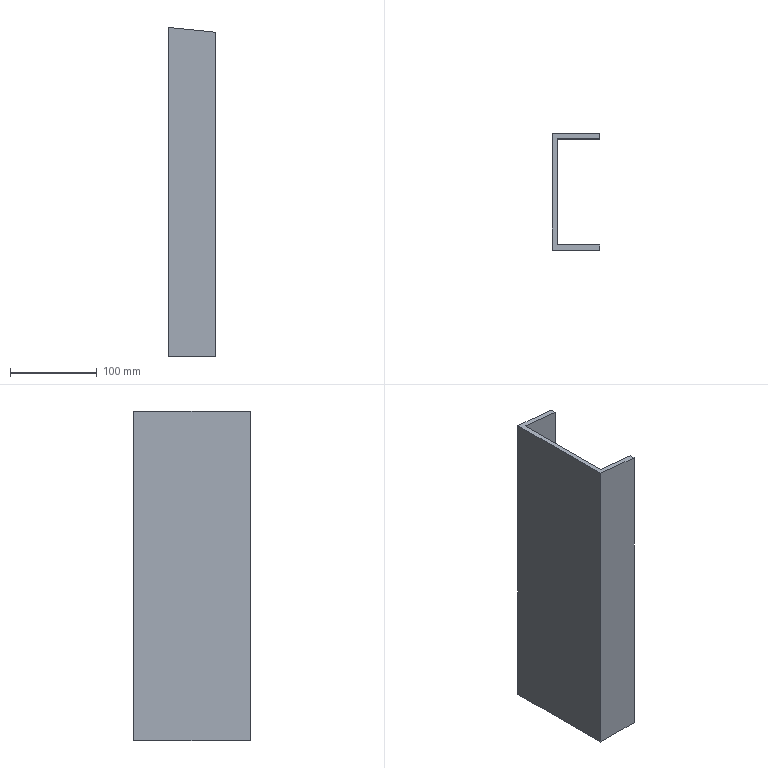Component | NX | RIGHT_FRAME450 | 1 solid | 10 faces | box 55 x 135 x 380.03 mm | volume 529247 mm3 | plane 10
STEP:
#1=CARTESIAN_POINT('',(0.,0.,0.));
#2=DIRECTION('',(0.,0.,1.));
#3=DIRECTION('',(1.,0.,0.));
#4=AXIS2_PLACEMENT_3D('',#1,#2,#3);
#5=CARTESIAN_POINT('',(1375.,1665.,380.029));
#6=VERTEX_POINT('',#5);
#7=CARTESIAN_POINT('',(1375.,1665.,-0.));
#8=VERTEX_POINT('',#7);
#9=CARTESIAN_POINT('',(1375.,1665.,400.));
#10=DIRECTION('',(0.,0.,-1.));
#11=VECTOR('',#10,1.);
#12=LINE('',#9,#11);
#13=CARTESIAN_POINT('',(1375.,1665.,400.));
#14=DIRECTION('',(-1.,0.,0.));
#15=DIRECTION('',(-0.,-1.,0.));
#16=AXIS2_PLACEMENT_3D('',#13,#14,#15);
#17=PLANE('',#16);
#18=CARTESIAN_POINT('',(0.,0.));
#19=DIRECTION('',(0.,-1.));
#20=VECTOR('',#19,1.);
#21=LINE('',#18,#20);
#22=(GEOMETRIC_REPRESENTATION_CONTEXT(2)PARAMETRIC_REPRESENTATION_CONTEXT()REPRESENTATION_CONTEXT('',''));
#23=DEFINITIONAL_REPRESENTATION('',(#21),#22);
#24=PCURVE('',#17,#23);
#25=CARTESIAN_POINT('',(1430.,1665.,400.));
#26=DIRECTION('',(0.,-1.,0.));
#27=DIRECTION('',(0.,0.,-1.));
#28=AXIS2_PLACEMENT_3D('',#25,#26,#27);
#29=PLANE('',#28);
#30=CARTESIAN_POINT('',(0.,-55.));
#31=DIRECTION('',(1.,0.));
#32=VECTOR('',#31,1.);
#33=LINE('',#30,#32);
#34=(GEOMETRIC_REPRESENTATION_CONTEXT(2)PARAMETRIC_REPRESENTATION_CONTEXT()REPRESENTATION_CONTEXT('',''));
#35=DEFINITIONAL_REPRESENTATION('',(#33),#34);
#36=PCURVE('',#29,#35);
#37=SURFACE_CURVE('',#12,(#24,#36),.PCURVE_S1.);
#38=EDGE_CURVE('',#6,#8,#37,.T.);
#39=ORIENTED_EDGE('',*,*,#38,.F.);
#40=CARTESIAN_POINT('',(1375.,1800.,380.029));
#41=VERTEX_POINT('',#40);
#42=CARTESIAN_POINT('',(1375.,1665.,380.029));
#43=DIRECTION('',(0.,1.,-0.));
#44=VECTOR('',#43,1.);
#45=LINE('',#42,#44);
#46=CARTESIAN_POINT('',(0.,-19.971));
#47=DIRECTION('',(-1.,-0.));
#48=VECTOR('',#47,1.);
#49=LINE('',#46,#48);
#50=(GEOMETRIC_REPRESENTATION_CONTEXT(2)PARAMETRIC_REPRESENTATION_CONTEXT()REPRESENTATION_CONTEXT('',''));
#51=DEFINITIONAL_REPRESENTATION('',(#49),#50);
#52=PCURVE('',#17,#51);
#53=CARTESIAN_POINT('',(1470.271,2035.,370.519));
#54=DIRECTION('',(0.09932,0.,0.9951));
#55=DIRECTION('',(0.9951,0.,-0.09932));
#56=AXIS2_PLACEMENT_3D('',#53,#54,#55);
#57=PLANE('',#56);
#58=CARTESIAN_POINT('',(-95.744,-370.));
#59=DIRECTION('',(0.,1.));
#60=VECTOR('',#59,1.);
#61=LINE('',#58,#60);
#62=(GEOMETRIC_REPRESENTATION_CONTEXT(2)PARAMETRIC_REPRESENTATION_CONTEXT()REPRESENTATION_CONTEXT('',''));
#63=DEFINITIONAL_REPRESENTATION('',(#61),#62);
#64=PCURVE('',#57,#63);
#65=SURFACE_CURVE('',#45,(#52,#64),.PCURVE_S1.);
#66=EDGE_CURVE('',#6,#41,#65,.T.);
#67=ORIENTED_EDGE('',*,*,#66,.T.);
#68=CARTESIAN_POINT('',(1375.,1800.,-0.));
#69=VERTEX_POINT('',#68);
#70=CARTESIAN_POINT('',(1375.,1800.,400.));
#71=DIRECTION('',(0.,0.,-1.));
#72=VECTOR('',#71,1.);
#73=LINE('',#70,#72);
#74=CARTESIAN_POINT('',(-135.,0.));
#75=DIRECTION('',(0.,-1.));
#76=VECTOR('',#75,1.);
#77=LINE('',#74,#76);
#78=(GEOMETRIC_REPRESENTATION_CONTEXT(2)PARAMETRIC_REPRESENTATION_CONTEXT()REPRESENTATION_CONTEXT('',''));
#79=DEFINITIONAL_REPRESENTATION('',(#77),#78);
#80=PCURVE('',#17,#79);
#81=CARTESIAN_POINT('',(1375.,1800.,400.));
#82=DIRECTION('',(0.,1.,0.));
#83=DIRECTION('',(0.,0.,1.));
#84=AXIS2_PLACEMENT_3D('',#81,#82,#83);
#85=PLANE('',#84);
#86=CARTESIAN_POINT('',(0.,0.));
#87=DIRECTION('',(-1.,0.));
#88=VECTOR('',#87,1.);
#89=LINE('',#86,#88);
#90=(GEOMETRIC_REPRESENTATION_CONTEXT(2)PARAMETRIC_REPRESENTATION_CONTEXT()REPRESENTATION_CONTEXT('',''));
#91=DEFINITIONAL_REPRESENTATION('',(#89),#90);
#92=PCURVE('',#85,#91);
#93=SURFACE_CURVE('',#73,(#80,#92),.PCURVE_S1.);
#94=EDGE_CURVE('',#41,#69,#93,.T.);
#95=ORIENTED_EDGE('',*,*,#94,.T.);
#96=CARTESIAN_POINT('',(1375.,1665.,-0.));
#97=DIRECTION('',(0.,1.,0.));
#98=VECTOR('',#97,1.);
#99=LINE('',#96,#98);
#100=CARTESIAN_POINT('',(0.,-400.));
#101=DIRECTION('',(-1.,0.));
#102=VECTOR('',#101,1.);
#103=LINE('',#100,#102);
#104=(GEOMETRIC_REPRESENTATION_CONTEXT(2)PARAMETRIC_REPRESENTATION_CONTEXT()REPRESENTATION_CONTEXT('',''));
#105=DEFINITIONAL_REPRESENTATION('',(#103),#104);
#106=PCURVE('',#17,#105);
#107=CARTESIAN_POINT('',(1375.,1800.,-0.));
#108=DIRECTION('',(0.,0.,-1.));
#109=DIRECTION('',(-1.,0.,0.));
#110=AXIS2_PLACEMENT_3D('',#107,#108,#109);
#111=PLANE('',#110);
#112=CARTESIAN_POINT('',(0.,-135.));
#113=DIRECTION('',(-0.,1.));
#114=VECTOR('',#113,1.);
#115=LINE('',#112,#114);
#116=(GEOMETRIC_REPRESENTATION_CONTEXT(2)PARAMETRIC_REPRESENTATION_CONTEXT()REPRESENTATION_CONTEXT('',''));
#117=DEFINITIONAL_REPRESENTATION('',(#115),#116);
#118=PCURVE('',#111,#117);
#119=SURFACE_CURVE('',#99,(#106,#118),.PCURVE_S1.);
#120=EDGE_CURVE('',#8,#69,#119,.T.);
#121=ORIENTED_EDGE('',*,*,#120,.F.);
#122=EDGE_LOOP('',(#39,#67,#95,#121));
#123=FACE_BOUND('',#122,.T.);
#124=ADVANCED_FACE('',(#123),#17,.T.);
#125=ORIENTED_EDGE('',*,*,#94,.F.);
#126=CARTESIAN_POINT('',(1430.,1800.,374.539));
#127=VERTEX_POINT('',#126);
#128=CARTESIAN_POINT('',(1373.026,1800.,380.226));
#129=DIRECTION('',(0.9951,0.,-0.09932));
#130=VECTOR('',#129,1.);
#131=LINE('',#128,#130);
#132=CARTESIAN_POINT('',(-19.774,-1.974));
#133=DIRECTION('',(-0.09932,0.9951));
#134=VECTOR('',#133,1.);
#135=LINE('',#132,#134);
#136=(GEOMETRIC_REPRESENTATION_CONTEXT(2)PARAMETRIC_REPRESENTATION_CONTEXT()REPRESENTATION_CONTEXT('',''));
#137=DEFINITIONAL_REPRESENTATION('',(#135),#136);
#138=PCURVE('',#85,#137);
#139=CARTESIAN_POINT('',(-97.728,-235.));
#140=DIRECTION('',(1.,0.));
#141=VECTOR('',#140,1.);
#142=LINE('',#139,#141);
#143=(GEOMETRIC_REPRESENTATION_CONTEXT(2)PARAMETRIC_REPRESENTATION_CONTEXT()REPRESENTATION_CONTEXT('',''));
#144=DEFINITIONAL_REPRESENTATION('',(#142),#143);
#145=PCURVE('',#57,#144);
#146=SURFACE_CURVE('',#131,(#138,#145),.PCURVE_S1.);
#147=EDGE_CURVE('',#41,#127,#146,.T.);
#148=ORIENTED_EDGE('',*,*,#147,.T.);
#149=CARTESIAN_POINT('',(1430.,1800.,-0.));
#150=VERTEX_POINT('',#149);
#151=CARTESIAN_POINT('',(1430.,1800.,400.));
#152=DIRECTION('',(0.,0.,-1.));
#153=VECTOR('',#152,1.);
#154=LINE('',#151,#153);
#155=CARTESIAN_POINT('',(0.,55.));
#156=DIRECTION('',(-1.,0.));
#157=VECTOR('',#156,1.);
#158=LINE('',#155,#157);
#159=(GEOMETRIC_REPRESENTATION_CONTEXT(2)PARAMETRIC_REPRESENTATION_CONTEXT()REPRESENTATION_CONTEXT('',''));
#160=DEFINITIONAL_REPRESENTATION('',(#158),#159);
#161=PCURVE('',#85,#160);
#162=CARTESIAN_POINT('',(1430.,1800.,400.));
#163=DIRECTION('',(1.,-0.,0.));
#164=DIRECTION('',(0.,1.,0.));
#165=AXIS2_PLACEMENT_3D('',#162,#163,#164);
#166=PLANE('',#165);
#167=CARTESIAN_POINT('',(0.,0.));
#168=DIRECTION('',(0.,-1.));
#169=VECTOR('',#168,1.);
#170=LINE('',#167,#169);
#171=(GEOMETRIC_REPRESENTATION_CONTEXT(2)PARAMETRIC_REPRESENTATION_CONTEXT()REPRESENTATION_CONTEXT('',''));
#172=DEFINITIONAL_REPRESENTATION('',(#170),#171);
#173=PCURVE('',#166,#172);
#174=SURFACE_CURVE('',#154,(#161,#173),.PCURVE_S1.);
#175=EDGE_CURVE('',#127,#150,#174,.T.);
#176=ORIENTED_EDGE('',*,*,#175,.T.);
#177=CARTESIAN_POINT('',(1375.,1800.,-0.));
#178=DIRECTION('',(1.,0.,0.));
#179=VECTOR('',#178,1.);
#180=LINE('',#177,#179);
#181=CARTESIAN_POINT('',(-400.,0.));
#182=DIRECTION('',(0.,1.));
#183=VECTOR('',#182,1.);
#184=LINE('',#181,#183);
#185=(GEOMETRIC_REPRESENTATION_CONTEXT(2)PARAMETRIC_REPRESENTATION_CONTEXT()REPRESENTATION_CONTEXT('',''));
#186=DEFINITIONAL_REPRESENTATION('',(#184),#185);
#187=PCURVE('',#85,#186);
#188=CARTESIAN_POINT('',(0.,0.));
#189=DIRECTION('',(-1.,0.));
#190=VECTOR('',#189,1.);
#191=LINE('',#188,#190);
#192=(GEOMETRIC_REPRESENTATION_CONTEXT(2)PARAMETRIC_REPRESENTATION_CONTEXT()REPRESENTATION_CONTEXT('',''));
#193=DEFINITIONAL_REPRESENTATION('',(#191),#192);
#194=PCURVE('',#111,#193);
#195=SURFACE_CURVE('',#180,(#187,#194),.PCURVE_S1.);
#196=EDGE_CURVE('',#69,#150,#195,.T.);
#197=ORIENTED_EDGE('',*,*,#196,.F.);
#198=EDGE_LOOP('',(#125,#148,#176,#197));
#199=FACE_BOUND('',#198,.T.);
#200=ADVANCED_FACE('',(#199),#85,.T.);
#201=ORIENTED_EDGE('',*,*,#175,.F.);
#202=CARTESIAN_POINT('',(1430.,1794.,374.539));
#203=VERTEX_POINT('',#202);
#204=CARTESIAN_POINT('',(1430.,1800.,374.539));
#205=DIRECTION('',(-0.,-1.,0.));
#206=VECTOR('',#205,1.);
#207=LINE('',#204,#206);
#208=CARTESIAN_POINT('',(0.,-25.461));
#209=DIRECTION('',(-1.,0.));
#210=VECTOR('',#209,1.);
#211=LINE('',#208,#210);
#212=(GEOMETRIC_REPRESENTATION_CONTEXT(2)PARAMETRIC_REPRESENTATION_CONTEXT()REPRESENTATION_CONTEXT('',''));
#213=DEFINITIONAL_REPRESENTATION('',(#211),#212);
#214=PCURVE('',#166,#213);
#215=CARTESIAN_POINT('',(-40.471,-235.));
#216=DIRECTION('',(-0.,-1.));
#217=VECTOR('',#216,1.);
#218=LINE('',#215,#217);
#219=(GEOMETRIC_REPRESENTATION_CONTEXT(2)PARAMETRIC_REPRESENTATION_CONTEXT()REPRESENTATION_CONTEXT('',''));
#220=DEFINITIONAL_REPRESENTATION('',(#218),#219);
#221=PCURVE('',#57,#220);
#222=SURFACE_CURVE('',#207,(#214,#221),.PCURVE_S1.);
#223=EDGE_CURVE('',#127,#203,#222,.T.);
#224=ORIENTED_EDGE('',*,*,#223,.T.);
#225=CARTESIAN_POINT('',(1430.,1794.,-0.));
#226=VERTEX_POINT('',#225);
#227=CARTESIAN_POINT('',(1430.,1794.,400.));
#228=DIRECTION('',(0.,0.,-1.));
#229=VECTOR('',#228,1.);
#230=LINE('',#227,#229);
#231=CARTESIAN_POINT('',(-6.,0.));
#232=DIRECTION('',(0.,-1.));
#233=VECTOR('',#232,1.);
#234=LINE('',#231,#233);
#235=(GEOMETRIC_REPRESENTATION_CONTEXT(2)PARAMETRIC_REPRESENTATION_CONTEXT()REPRESENTATION_CONTEXT('',''));
#236=DEFINITIONAL_REPRESENTATION('',(#234),#235);
#237=PCURVE('',#166,#236);
#238=CARTESIAN_POINT('',(1430.,1794.,400.));
#239=DIRECTION('',(-0.,-1.,0.));
#240=DIRECTION('',(1.,-0.,0.));
#241=AXIS2_PLACEMENT_3D('',#238,#239,#240);
#242=PLANE('',#241);
#243=CARTESIAN_POINT('',(0.,0.));
#244=DIRECTION('',(0.,-1.));
#245=VECTOR('',#244,1.);
#246=LINE('',#243,#245);
#247=(GEOMETRIC_REPRESENTATION_CONTEXT(2)PARAMETRIC_REPRESENTATION_CONTEXT()REPRESENTATION_CONTEXT('',''));
#248=DEFINITIONAL_REPRESENTATION('',(#246),#247);
#249=PCURVE('',#242,#248);
#250=SURFACE_CURVE('',#230,(#237,#249),.PCURVE_S1.);
#251=EDGE_CURVE('',#203,#226,#250,.T.);
#252=ORIENTED_EDGE('',*,*,#251,.T.);
#253=CARTESIAN_POINT('',(1430.,1800.,-0.));
#254=DIRECTION('',(-0.,-1.,0.));
#255=VECTOR('',#254,1.);
#256=LINE('',#253,#255);
#257=CARTESIAN_POINT('',(0.,-400.));
#258=DIRECTION('',(-1.,0.));
#259=VECTOR('',#258,1.);
#260=LINE('',#257,#259);
#261=(GEOMETRIC_REPRESENTATION_CONTEXT(2)PARAMETRIC_REPRESENTATION_CONTEXT()REPRESENTATION_CONTEXT('',''));
#262=DEFINITIONAL_REPRESENTATION('',(#260),#261);
#263=PCURVE('',#166,#262);
#264=CARTESIAN_POINT('',(-55.,0.));
#265=DIRECTION('',(0.,-1.));
#266=VECTOR('',#265,1.);
#267=LINE('',#264,#266);
#268=(GEOMETRIC_REPRESENTATION_CONTEXT(2)PARAMETRIC_REPRESENTATION_CONTEXT()REPRESENTATION_CONTEXT('',''));
#269=DEFINITIONAL_REPRESENTATION('',(#267),#268);
#270=PCURVE('',#111,#269);
#271=SURFACE_CURVE('',#256,(#263,#270),.PCURVE_S1.);
#272=EDGE_CURVE('',#150,#226,#271,.T.);
#273=ORIENTED_EDGE('',*,*,#272,.F.);
#274=EDGE_LOOP('',(#201,#224,#252,#273));
#275=FACE_BOUND('',#274,.T.);
#276=ADVANCED_FACE('',(#275),#166,.T.);
#277=ORIENTED_EDGE('',*,*,#251,.F.);
#278=CARTESIAN_POINT('',(1381.,1794.,379.43));
#279=VERTEX_POINT('',#278);
#280=CARTESIAN_POINT('',(1427.484,1794.,374.79));
#281=DIRECTION('',(-0.9951,0.,0.09932));
#282=VECTOR('',#281,1.);
#283=LINE('',#280,#282);
#284=CARTESIAN_POINT('',(-2.516,-25.21));
#285=DIRECTION('',(-0.9951,0.09932));
#286=VECTOR('',#285,1.);
#287=LINE('',#284,#286);
#288=(GEOMETRIC_REPRESENTATION_CONTEXT(2)PARAMETRIC_REPRESENTATION_CONTEXT()REPRESENTATION_CONTEXT('',''));
#289=DEFINITIONAL_REPRESENTATION('',(#287),#288);
#290=PCURVE('',#242,#289);
#291=CARTESIAN_POINT('',(-43.,-241.));
#292=DIRECTION('',(-1.,0.));
#293=VECTOR('',#292,1.);
#294=LINE('',#291,#293);
#295=(GEOMETRIC_REPRESENTATION_CONTEXT(2)PARAMETRIC_REPRESENTATION_CONTEXT()REPRESENTATION_CONTEXT('',''));
#296=DEFINITIONAL_REPRESENTATION('',(#294),#295);
#297=PCURVE('',#57,#296);
#298=SURFACE_CURVE('',#283,(#290,#297),.PCURVE_S1.);
#299=EDGE_CURVE('',#203,#279,#298,.T.);
#300=ORIENTED_EDGE('',*,*,#299,.T.);
#301=CARTESIAN_POINT('',(1381.,1794.,-0.));
#302=VERTEX_POINT('',#301);
#303=CARTESIAN_POINT('',(1381.,1794.,400.));
#304=DIRECTION('',(0.,0.,-1.));
#305=VECTOR('',#304,1.);
#306=LINE('',#303,#305);
#307=CARTESIAN_POINT('',(-49.,0.));
#308=DIRECTION('',(0.,-1.));
#309=VECTOR('',#308,1.);
#310=LINE('',#307,#309);
#311=(GEOMETRIC_REPRESENTATION_CONTEXT(2)PARAMETRIC_REPRESENTATION_CONTEXT()REPRESENTATION_CONTEXT('',''));
#312=DEFINITIONAL_REPRESENTATION('',(#310),#311);
#313=PCURVE('',#242,#312);
#314=CARTESIAN_POINT('',(1381.,1794.,400.));
#315=DIRECTION('',(1.,-0.,0.));
#316=DIRECTION('',(0.,1.,0.));
#317=AXIS2_PLACEMENT_3D('',#314,#315,#316);
#318=PLANE('',#317);
#319=CARTESIAN_POINT('',(0.,0.));
#320=DIRECTION('',(0.,-1.));
#321=VECTOR('',#320,1.);
#322=LINE('',#319,#321);
#323=(GEOMETRIC_REPRESENTATION_CONTEXT(2)PARAMETRIC_REPRESENTATION_CONTEXT()REPRESENTATION_CONTEXT('',''));
#324=DEFINITIONAL_REPRESENTATION('',(#322),#323);
#325=PCURVE('',#318,#324);
#326=SURFACE_CURVE('',#306,(#313,#325),.PCURVE_S1.);
#327=EDGE_CURVE('',#279,#302,#326,.T.);
#328=ORIENTED_EDGE('',*,*,#327,.T.);
#329=CARTESIAN_POINT('',(1430.,1794.,-0.));
#330=DIRECTION('',(-1.,0.,0.));
#331=VECTOR('',#330,1.);
#332=LINE('',#329,#331);
#333=CARTESIAN_POINT('',(0.,-400.));
#334=DIRECTION('',(-1.,0.));
#335=VECTOR('',#334,1.);
#336=LINE('',#333,#335);
#337=(GEOMETRIC_REPRESENTATION_CONTEXT(2)PARAMETRIC_REPRESENTATION_CONTEXT()REPRESENTATION_CONTEXT('',''));
#338=DEFINITIONAL_REPRESENTATION('',(#336),#337);
#339=PCURVE('',#242,#338);
#340=CARTESIAN_POINT('',(-55.,-6.));
#341=DIRECTION('',(1.,0.));
#342=VECTOR('',#341,1.);
#343=LINE('',#340,#342);
#344=(GEOMETRIC_REPRESENTATION_CONTEXT(2)PARAMETRIC_REPRESENTATION_CONTEXT()REPRESENTATION_CONTEXT('',''));
#345=DEFINITIONAL_REPRESENTATION('',(#343),#344);
#346=PCURVE('',#111,#345);
#347=SURFACE_CURVE('',#332,(#339,#346),.PCURVE_S1.);
#348=EDGE_CURVE('',#226,#302,#347,.T.);
#349=ORIENTED_EDGE('',*,*,#348,.F.);
#350=EDGE_LOOP('',(#277,#300,#328,#349));
#351=FACE_BOUND('',#350,.T.);
#352=ADVANCED_FACE('',(#351),#242,.T.);
#353=ORIENTED_EDGE('',*,*,#327,.F.);
#354=CARTESIAN_POINT('',(1381.,1671.,379.43));
#355=VERTEX_POINT('',#354);
#356=CARTESIAN_POINT('',(1381.,1794.,379.43));
#357=DIRECTION('',(-0.,-1.,0.));
#358=VECTOR('',#357,1.);
#359=LINE('',#356,#358);
#360=CARTESIAN_POINT('',(0.,-20.57));
#361=DIRECTION('',(-1.,0.));
#362=VECTOR('',#361,1.);
#363=LINE('',#360,#362);
#364=(GEOMETRIC_REPRESENTATION_CONTEXT(2)PARAMETRIC_REPRESENTATION_CONTEXT()REPRESENTATION_CONTEXT('',''));
#365=DEFINITIONAL_REPRESENTATION('',(#363),#364);
#366=PCURVE('',#318,#365);
#367=CARTESIAN_POINT('',(-89.715,-241.));
#368=DIRECTION('',(-0.,-1.));
#369=VECTOR('',#368,1.);
#370=LINE('',#367,#369);
#371=(GEOMETRIC_REPRESENTATION_CONTEXT(2)PARAMETRIC_REPRESENTATION_CONTEXT()REPRESENTATION_CONTEXT('',''));
#372=DEFINITIONAL_REPRESENTATION('',(#370),#371);
#373=PCURVE('',#57,#372);
#374=SURFACE_CURVE('',#359,(#366,#373),.PCURVE_S1.);
#375=EDGE_CURVE('',#279,#355,#374,.T.);
#376=ORIENTED_EDGE('',*,*,#375,.T.);
#377=CARTESIAN_POINT('',(1381.,1671.,-0.));
#378=VERTEX_POINT('',#377);
#379=CARTESIAN_POINT('',(1381.,1671.,400.));
#380=DIRECTION('',(0.,0.,-1.));
#381=VECTOR('',#380,1.);
#382=LINE('',#379,#381);
#383=CARTESIAN_POINT('',(-123.,0.));
#384=DIRECTION('',(0.,-1.));
#385=VECTOR('',#384,1.);
#386=LINE('',#383,#385);
#387=(GEOMETRIC_REPRESENTATION_CONTEXT(2)PARAMETRIC_REPRESENTATION_CONTEXT()REPRESENTATION_CONTEXT('',''));
#388=DEFINITIONAL_REPRESENTATION('',(#386),#387);
#389=PCURVE('',#318,#388);
#390=CARTESIAN_POINT('',(1381.,1671.,400.));
#391=DIRECTION('',(0.,1.,0.));
#392=DIRECTION('',(-1.,0.,0.));
#393=AXIS2_PLACEMENT_3D('',#390,#391,#392);
#394=PLANE('',#393);
#395=CARTESIAN_POINT('',(0.,0.));
#396=DIRECTION('',(0.,-1.));
#397=VECTOR('',#396,1.);
#398=LINE('',#395,#397);
#399=(GEOMETRIC_REPRESENTATION_CONTEXT(2)PARAMETRIC_REPRESENTATION_CONTEXT()REPRESENTATION_CONTEXT('',''));
#400=DEFINITIONAL_REPRESENTATION('',(#398),#399);
#401=PCURVE('',#394,#400);
#402=SURFACE_CURVE('',#382,(#389,#401),.PCURVE_S1.);
#403=EDGE_CURVE('',#355,#378,#402,.T.);
#404=ORIENTED_EDGE('',*,*,#403,.T.);
#405=CARTESIAN_POINT('',(1381.,1794.,-0.));
#406=DIRECTION('',(-0.,-1.,0.));
#407=VECTOR('',#406,1.);
#408=LINE('',#405,#407);
#409=CARTESIAN_POINT('',(0.,-400.));
#410=DIRECTION('',(-1.,0.));
#411=VECTOR('',#410,1.);
#412=LINE('',#409,#411);
#413=(GEOMETRIC_REPRESENTATION_CONTEXT(2)PARAMETRIC_REPRESENTATION_CONTEXT()REPRESENTATION_CONTEXT('',''));
#414=DEFINITIONAL_REPRESENTATION('',(#412),#413);
#415=PCURVE('',#318,#414);
#416=CARTESIAN_POINT('',(-6.,-6.));
#417=DIRECTION('',(0.,-1.));
#418=VECTOR('',#417,1.);
#419=LINE('',#416,#418);
#420=(GEOMETRIC_REPRESENTATION_CONTEXT(2)PARAMETRIC_REPRESENTATION_CONTEXT()REPRESENTATION_CONTEXT('',''));
#421=DEFINITIONAL_REPRESENTATION('',(#419),#420);
#422=PCURVE('',#111,#421);
#423=SURFACE_CURVE('',#408,(#415,#422),.PCURVE_S1.);
#424=EDGE_CURVE('',#302,#378,#423,.T.);
#425=ORIENTED_EDGE('',*,*,#424,.F.);
#426=EDGE_LOOP('',(#353,#376,#404,#425));
#427=FACE_BOUND('',#426,.T.);
#428=ADVANCED_FACE('',(#427),#318,.T.);
#429=ORIENTED_EDGE('',*,*,#403,.F.);
#430=CARTESIAN_POINT('',(1430.,1671.,374.539));
#431=VERTEX_POINT('',#430);
#432=CARTESIAN_POINT('',(1378.967,1671.,379.633));
#433=DIRECTION('',(0.9951,-0.,-0.09932));
#434=VECTOR('',#433,1.);
#435=LINE('',#432,#434);
#436=CARTESIAN_POINT('',(2.033,-20.367));
#437=DIRECTION('',(-0.9951,-0.09932));
#438=VECTOR('',#437,1.);
#439=LINE('',#436,#438);
#440=(GEOMETRIC_REPRESENTATION_CONTEXT(2)PARAMETRIC_REPRESENTATION_CONTEXT()REPRESENTATION_CONTEXT('',''));
#441=DEFINITIONAL_REPRESENTATION('',(#439),#440);
#442=PCURVE('',#394,#441);
#443=CARTESIAN_POINT('',(-91.758,-364.));
#444=DIRECTION('',(1.,-0.));
#445=VECTOR('',#444,1.);
#446=LINE('',#443,#445);
#447=(GEOMETRIC_REPRESENTATION_CONTEXT(2)PARAMETRIC_REPRESENTATION_CONTEXT()REPRESENTATION_CONTEXT('',''));
#448=DEFINITIONAL_REPRESENTATION('',(#446),#447);
#449=PCURVE('',#57,#448);
#450=SURFACE_CURVE('',#435,(#442,#449),.PCURVE_S1.);
#451=EDGE_CURVE('',#355,#431,#450,.T.);
#452=ORIENTED_EDGE('',*,*,#451,.T.);
#453=CARTESIAN_POINT('',(1430.,1671.,-0.));
#454=VERTEX_POINT('',#453);
#455=CARTESIAN_POINT('',(1430.,1671.,400.));
#456=DIRECTION('',(0.,0.,-1.));
#457=VECTOR('',#456,1.);
#458=LINE('',#455,#457);
#459=CARTESIAN_POINT('',(-49.,0.));
#460=DIRECTION('',(0.,-1.));
#461=VECTOR('',#460,1.);
#462=LINE('',#459,#461);
#463=(GEOMETRIC_REPRESENTATION_CONTEXT(2)PARAMETRIC_REPRESENTATION_CONTEXT()REPRESENTATION_CONTEXT('',''));
#464=DEFINITIONAL_REPRESENTATION('',(#462),#463);
#465=PCURVE('',#394,#464);
#466=CARTESIAN_POINT('',(1430.,1671.,400.));
#467=DIRECTION('',(1.,0.,0.));
#468=DIRECTION('',(0.,0.,-1.));
#469=AXIS2_PLACEMENT_3D('',#466,#467,#468);
#470=PLANE('',#469);
#471=CARTESIAN_POINT('',(0.,0.));
#472=DIRECTION('',(1.,0.));
#473=VECTOR('',#472,1.);
#474=LINE('',#471,#473);
#475=(GEOMETRIC_REPRESENTATION_CONTEXT(2)PARAMETRIC_REPRESENTATION_CONTEXT()REPRESENTATION_CONTEXT('',''));
#476=DEFINITIONAL_REPRESENTATION('',(#474),#475);
#477=PCURVE('',#470,#476);
#478=SURFACE_CURVE('',#458,(#465,#477),.PCURVE_S1.);
#479=EDGE_CURVE('',#431,#454,#478,.T.);
#480=ORIENTED_EDGE('',*,*,#479,.T.);
#481=CARTESIAN_POINT('',(1381.,1671.,-0.));
#482=DIRECTION('',(1.,-0.,0.));
#483=VECTOR('',#482,1.);
#484=LINE('',#481,#483);
#485=CARTESIAN_POINT('',(0.,-400.));
#486=DIRECTION('',(-1.,0.));
#487=VECTOR('',#486,1.);
#488=LINE('',#485,#487);
#489=(GEOMETRIC_REPRESENTATION_CONTEXT(2)PARAMETRIC_REPRESENTATION_CONTEXT()REPRESENTATION_CONTEXT('',''));
#490=DEFINITIONAL_REPRESENTATION('',(#488),#489);
#491=PCURVE('',#394,#490);
#492=CARTESIAN_POINT('',(-6.,-129.));
#493=DIRECTION('',(-1.,-0.));
#494=VECTOR('',#493,1.);
#495=LINE('',#492,#494);
#496=(GEOMETRIC_REPRESENTATION_CONTEXT(2)PARAMETRIC_REPRESENTATION_CONTEXT()REPRESENTATION_CONTEXT('',''));
#497=DEFINITIONAL_REPRESENTATION('',(#495),#496);
#498=PCURVE('',#111,#497);
#499=SURFACE_CURVE('',#484,(#491,#498),.PCURVE_S1.);
#500=EDGE_CURVE('',#378,#454,#499,.T.);
#501=ORIENTED_EDGE('',*,*,#500,.F.);
#502=EDGE_LOOP('',(#429,#452,#480,#501));
#503=FACE_BOUND('',#502,.T.);
#504=ADVANCED_FACE('',(#503),#394,.T.);
#505=ORIENTED_EDGE('',*,*,#479,.F.);
#506=CARTESIAN_POINT('',(1430.,1665.,374.539));
#507=VERTEX_POINT('',#506);
#508=CARTESIAN_POINT('',(1430.,1671.,374.539));
#509=DIRECTION('',(0.,-1.,0.));
#510=VECTOR('',#509,1.);
#511=LINE('',#508,#510);
#512=CARTESIAN_POINT('',(25.461,0.));
#513=DIRECTION('',(0.,-1.));
#514=VECTOR('',#513,1.);
#515=LINE('',#512,#514);
#516=(GEOMETRIC_REPRESENTATION_CONTEXT(2)PARAMETRIC_REPRESENTATION_CONTEXT()REPRESENTATION_CONTEXT('',''));
#517=DEFINITIONAL_REPRESENTATION('',(#515),#516);
#518=PCURVE('',#470,#517);
#519=CARTESIAN_POINT('',(-40.471,-364.));
#520=DIRECTION('',(0.,-1.));
#521=VECTOR('',#520,1.);
#522=LINE('',#519,#521);
#523=(GEOMETRIC_REPRESENTATION_CONTEXT(2)PARAMETRIC_REPRESENTATION_CONTEXT()REPRESENTATION_CONTEXT('',''));
#524=DEFINITIONAL_REPRESENTATION('',(#522),#523);
#525=PCURVE('',#57,#524);
#526=SURFACE_CURVE('',#511,(#518,#525),.PCURVE_S1.);
#527=EDGE_CURVE('',#431,#507,#526,.T.);
#528=ORIENTED_EDGE('',*,*,#527,.T.);
#529=CARTESIAN_POINT('',(1430.,1665.,-0.));
#530=VERTEX_POINT('',#529);
#531=CARTESIAN_POINT('',(1430.,1665.,400.));
#532=DIRECTION('',(0.,0.,-1.));
#533=VECTOR('',#532,1.);
#534=LINE('',#531,#533);
#535=CARTESIAN_POINT('',(0.,-6.));
#536=DIRECTION('',(1.,0.));
#537=VECTOR('',#536,1.);
#538=LINE('',#535,#537);
#539=(GEOMETRIC_REPRESENTATION_CONTEXT(2)PARAMETRIC_REPRESENTATION_CONTEXT()REPRESENTATION_CONTEXT('',''));
#540=DEFINITIONAL_REPRESENTATION('',(#538),#539);
#541=PCURVE('',#470,#540);
#542=CARTESIAN_POINT('',(0.,0.));
#543=DIRECTION('',(1.,0.));
#544=VECTOR('',#543,1.);
#545=LINE('',#542,#544);
#546=(GEOMETRIC_REPRESENTATION_CONTEXT(2)PARAMETRIC_REPRESENTATION_CONTEXT()REPRESENTATION_CONTEXT('',''));
#547=DEFINITIONAL_REPRESENTATION('',(#545),#546);
#548=PCURVE('',#29,#547);
#549=SURFACE_CURVE('',#534,(#541,#548),.PCURVE_S1.);
#550=EDGE_CURVE('',#507,#530,#549,.T.);
#551=ORIENTED_EDGE('',*,*,#550,.T.);
#552=CARTESIAN_POINT('',(1430.,1671.,-0.));
#553=DIRECTION('',(0.,-1.,0.));
#554=VECTOR('',#553,1.);
#555=LINE('',#552,#554);
#556=CARTESIAN_POINT('',(400.,0.));
#557=DIRECTION('',(0.,-1.));
#558=VECTOR('',#557,1.);
#559=LINE('',#556,#558);
#560=(GEOMETRIC_REPRESENTATION_CONTEXT(2)PARAMETRIC_REPRESENTATION_CONTEXT()REPRESENTATION_CONTEXT('',''));
#561=DEFINITIONAL_REPRESENTATION('',(#559),#560);
#562=PCURVE('',#470,#561);
#563=CARTESIAN_POINT('',(-55.,-129.));
#564=DIRECTION('',(0.,-1.));
#565=VECTOR('',#564,1.);
#566=LINE('',#563,#565);
#567=(GEOMETRIC_REPRESENTATION_CONTEXT(2)PARAMETRIC_REPRESENTATION_CONTEXT()REPRESENTATION_CONTEXT('',''));
#568=DEFINITIONAL_REPRESENTATION('',(#566),#567);
#569=PCURVE('',#111,#568);
#570=SURFACE_CURVE('',#555,(#562,#569),.PCURVE_S1.);
#571=EDGE_CURVE('',#454,#530,#570,.T.);
#572=ORIENTED_EDGE('',*,*,#571,.F.);
#573=EDGE_LOOP('',(#505,#528,#551,#572));
#574=FACE_BOUND('',#573,.T.);
#575=ADVANCED_FACE('',(#574),#470,.T.);
#576=ORIENTED_EDGE('',*,*,#550,.F.);
#577=CARTESIAN_POINT('',(1470.271,1665.,370.519));
#578=DIRECTION('',(-0.9951,0.,0.09932));
#579=VECTOR('',#578,1.);
#580=LINE('',#577,#579);
#581=CARTESIAN_POINT('',(29.481,40.271));
#582=DIRECTION('',(-0.09932,-0.9951));
#583=VECTOR('',#582,1.);
#584=LINE('',#581,#583);
#585=(GEOMETRIC_REPRESENTATION_CONTEXT(2)PARAMETRIC_REPRESENTATION_CONTEXT()REPRESENTATION_CONTEXT('',''));
#586=DEFINITIONAL_REPRESENTATION('',(#584),#585);
#587=PCURVE('',#29,#586);
#588=CARTESIAN_POINT('',(0.,-370.));
#589=DIRECTION('',(-1.,0.));
#590=VECTOR('',#589,1.);
#591=LINE('',#588,#590);
#592=(GEOMETRIC_REPRESENTATION_CONTEXT(2)PARAMETRIC_REPRESENTATION_CONTEXT()REPRESENTATION_CONTEXT('',''));
#593=DEFINITIONAL_REPRESENTATION('',(#591),#592);
#594=PCURVE('',#57,#593);
#595=SURFACE_CURVE('',#580,(#587,#594),.PCURVE_S1.);
#596=EDGE_CURVE('',#507,#6,#595,.T.);
#597=ORIENTED_EDGE('',*,*,#596,.T.);
#598=ORIENTED_EDGE('',*,*,#38,.T.);
#599=CARTESIAN_POINT('',(1430.,1665.,-0.));
#600=DIRECTION('',(-1.,0.,0.));
#601=VECTOR('',#600,1.);
#602=LINE('',#599,#601);
#603=CARTESIAN_POINT('',(400.,0.));
#604=DIRECTION('',(0.,-1.));
#605=VECTOR('',#604,1.);
#606=LINE('',#603,#605);
#607=(GEOMETRIC_REPRESENTATION_CONTEXT(2)PARAMETRIC_REPRESENTATION_CONTEXT()REPRESENTATION_CONTEXT('',''));
#608=DEFINITIONAL_REPRESENTATION('',(#606),#607);
#609=PCURVE('',#29,#608);
#610=CARTESIAN_POINT('',(-55.,-135.));
#611=DIRECTION('',(1.,0.));
#612=VECTOR('',#611,1.);
#613=LINE('',#610,#612);
#614=(GEOMETRIC_REPRESENTATION_CONTEXT(2)PARAMETRIC_REPRESENTATION_CONTEXT()REPRESENTATION_CONTEXT('',''));
#615=DEFINITIONAL_REPRESENTATION('',(#613),#614);
#616=PCURVE('',#111,#615);
#617=SURFACE_CURVE('',#602,(#609,#616),.PCURVE_S1.);
#618=EDGE_CURVE('',#530,#8,#617,.T.);
#619=ORIENTED_EDGE('',*,*,#618,.F.);
#620=EDGE_LOOP('',(#576,#597,#598,#619));
#621=FACE_BOUND('',#620,.T.);
#622=ADVANCED_FACE('',(#621),#29,.T.);
#623=ORIENTED_EDGE('',*,*,#120,.T.);
#624=ORIENTED_EDGE('',*,*,#196,.T.);
#625=ORIENTED_EDGE('',*,*,#272,.T.);
#626=ORIENTED_EDGE('',*,*,#348,.T.);
#627=ORIENTED_EDGE('',*,*,#424,.T.);
#628=ORIENTED_EDGE('',*,*,#500,.T.);
#629=ORIENTED_EDGE('',*,*,#571,.T.);
#630=ORIENTED_EDGE('',*,*,#618,.T.);
#631=EDGE_LOOP('',(#623,#624,#625,#626,#627,#628,#629,#630));
#632=FACE_BOUND('',#631,.T.);
#633=ADVANCED_FACE('',(#632),#111,.T.);
#634=ORIENTED_EDGE('',*,*,#596,.F.);
#635=ORIENTED_EDGE('',*,*,#527,.F.);
#636=ORIENTED_EDGE('',*,*,#451,.F.);
#637=ORIENTED_EDGE('',*,*,#375,.F.);
#638=ORIENTED_EDGE('',*,*,#299,.F.);
#639=ORIENTED_EDGE('',*,*,#223,.F.);
#640=ORIENTED_EDGE('',*,*,#147,.F.);
#641=ORIENTED_EDGE('',*,*,#66,.F.);
#642=EDGE_LOOP('',(#634,#635,#636,#637,#638,#639,#640,#641));
#643=FACE_BOUND('',#642,.T.);
#644=ADVANCED_FACE('',(#643),#57,.T.);
#645=CLOSED_SHELL('',(#124,#200,#276,#352,#428,#504,#575,#622,#633,#644));
#646=MANIFOLD_SOLID_BREP('',#645);
#647=(LENGTH_UNIT()NAMED_UNIT(*)SI_UNIT(.MILLI.,.METRE.));
#648=UNCERTAINTY_MEASURE_WITH_UNIT(LENGTH_MEASURE(0.0000001),#647,'','');
#649=(NAMED_UNIT(*)PLANE_ANGLE_UNIT()SI_UNIT($,.RADIAN.));
#650=(NAMED_UNIT(*)SI_UNIT($,.STERADIAN.)SOLID_ANGLE_UNIT());
#651=(GEOMETRIC_REPRESENTATION_CONTEXT(3)GLOBAL_UNCERTAINTY_ASSIGNED_CONTEXT((#648))GLOBAL_UNIT_ASSIGNED_CONTEXT((#647,#649,#650))REPRESENTATION_CONTEXT('',''));
#652=ADVANCED_BREP_SHAPE_REPRESENTATION('',(#4,#646),#651);